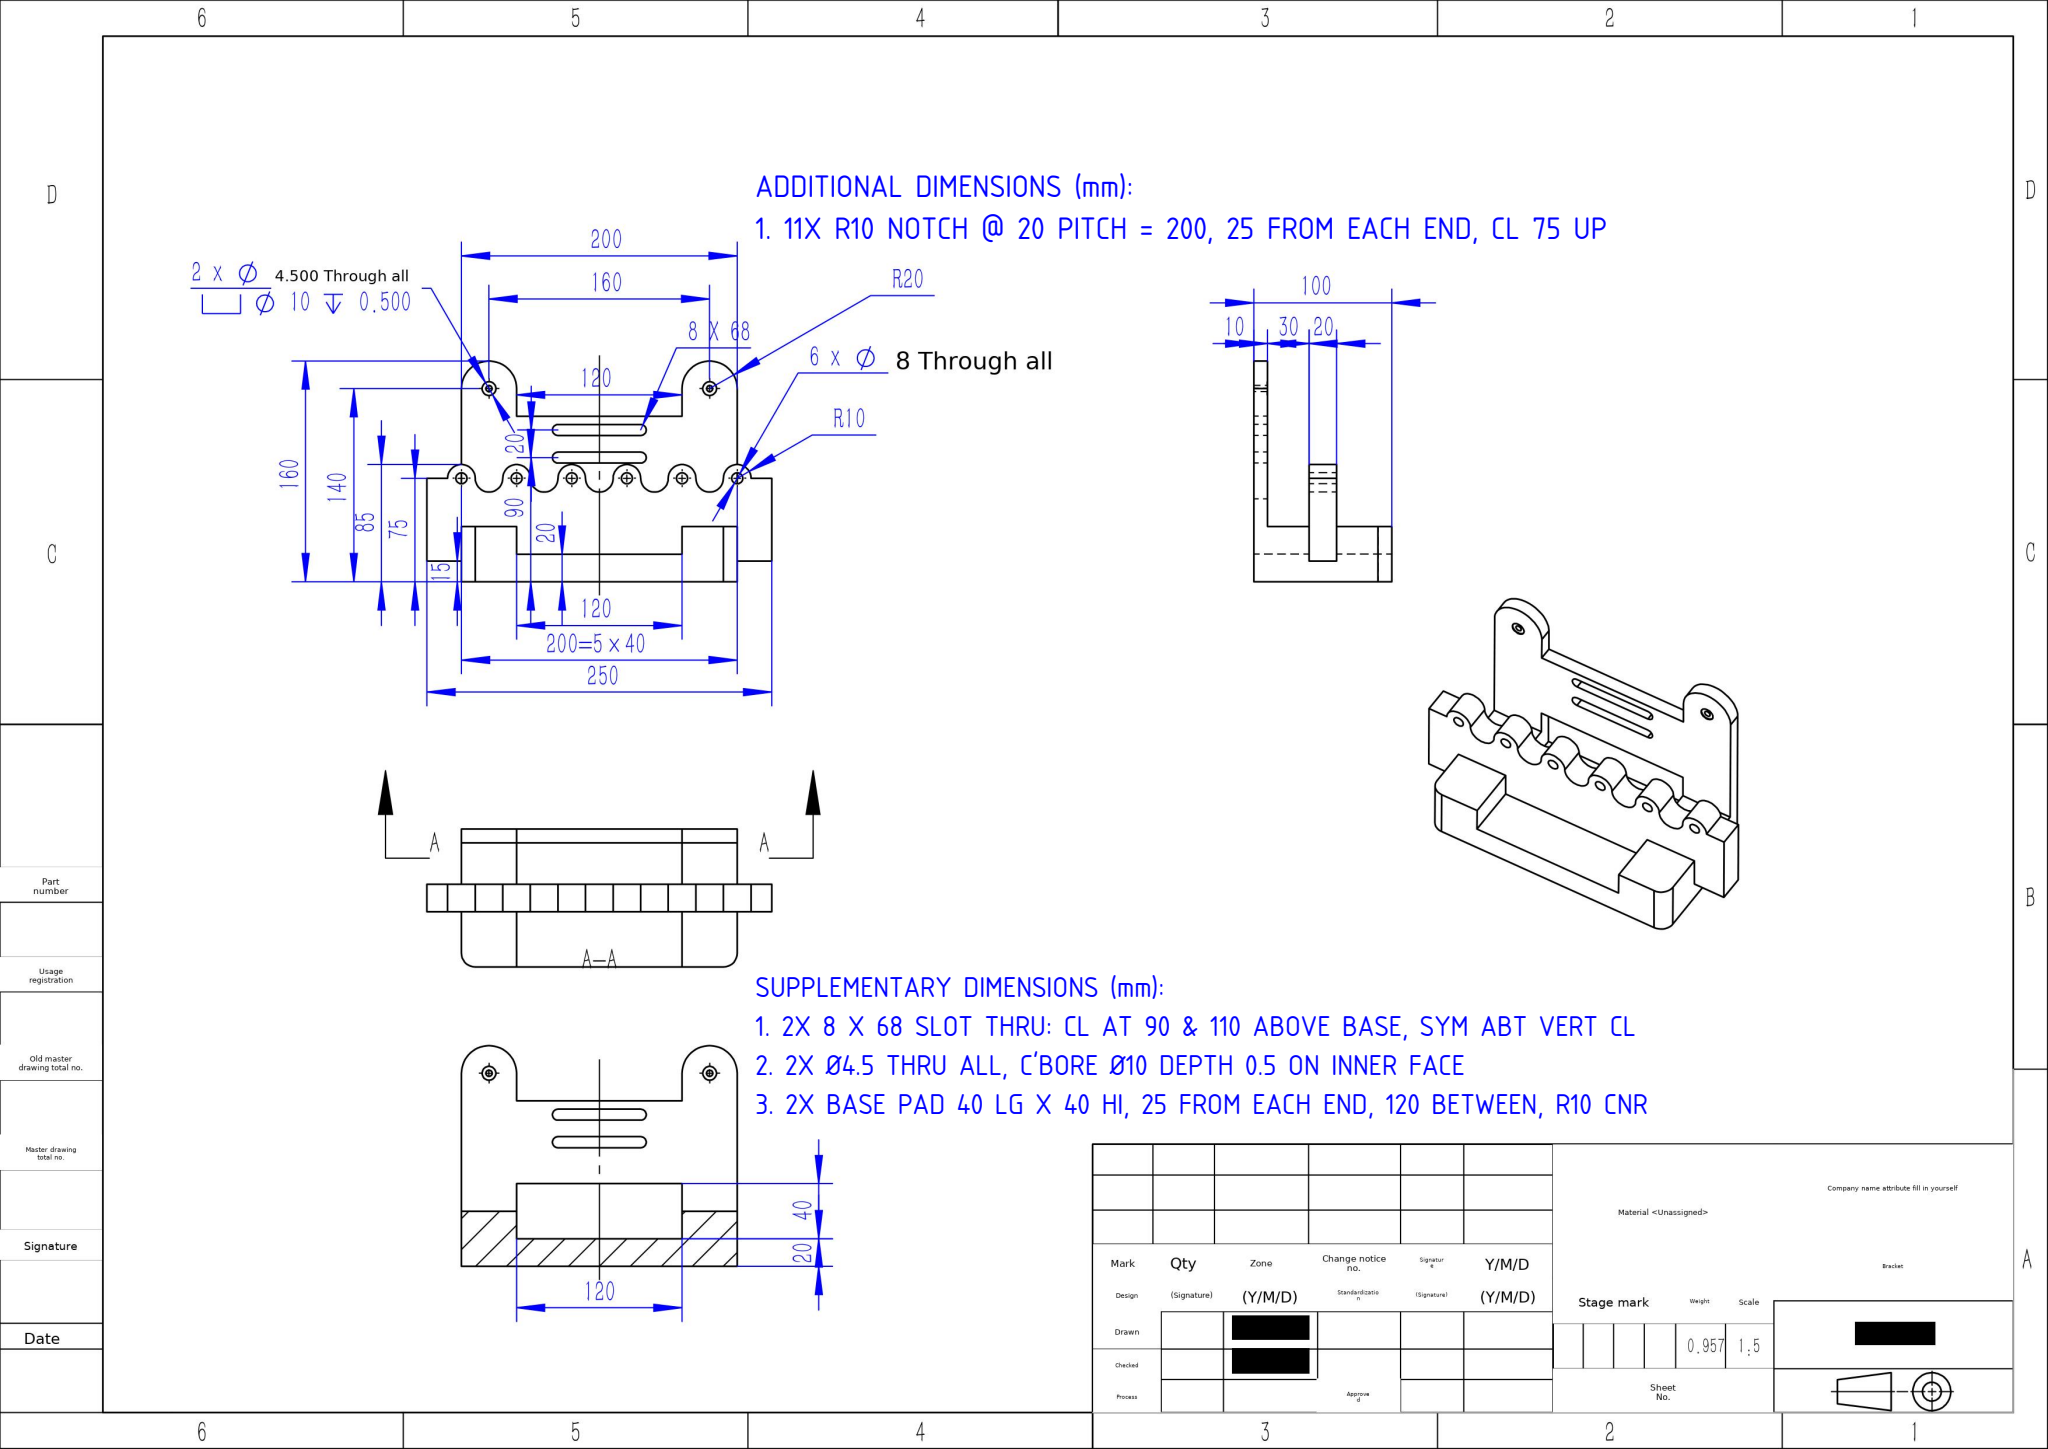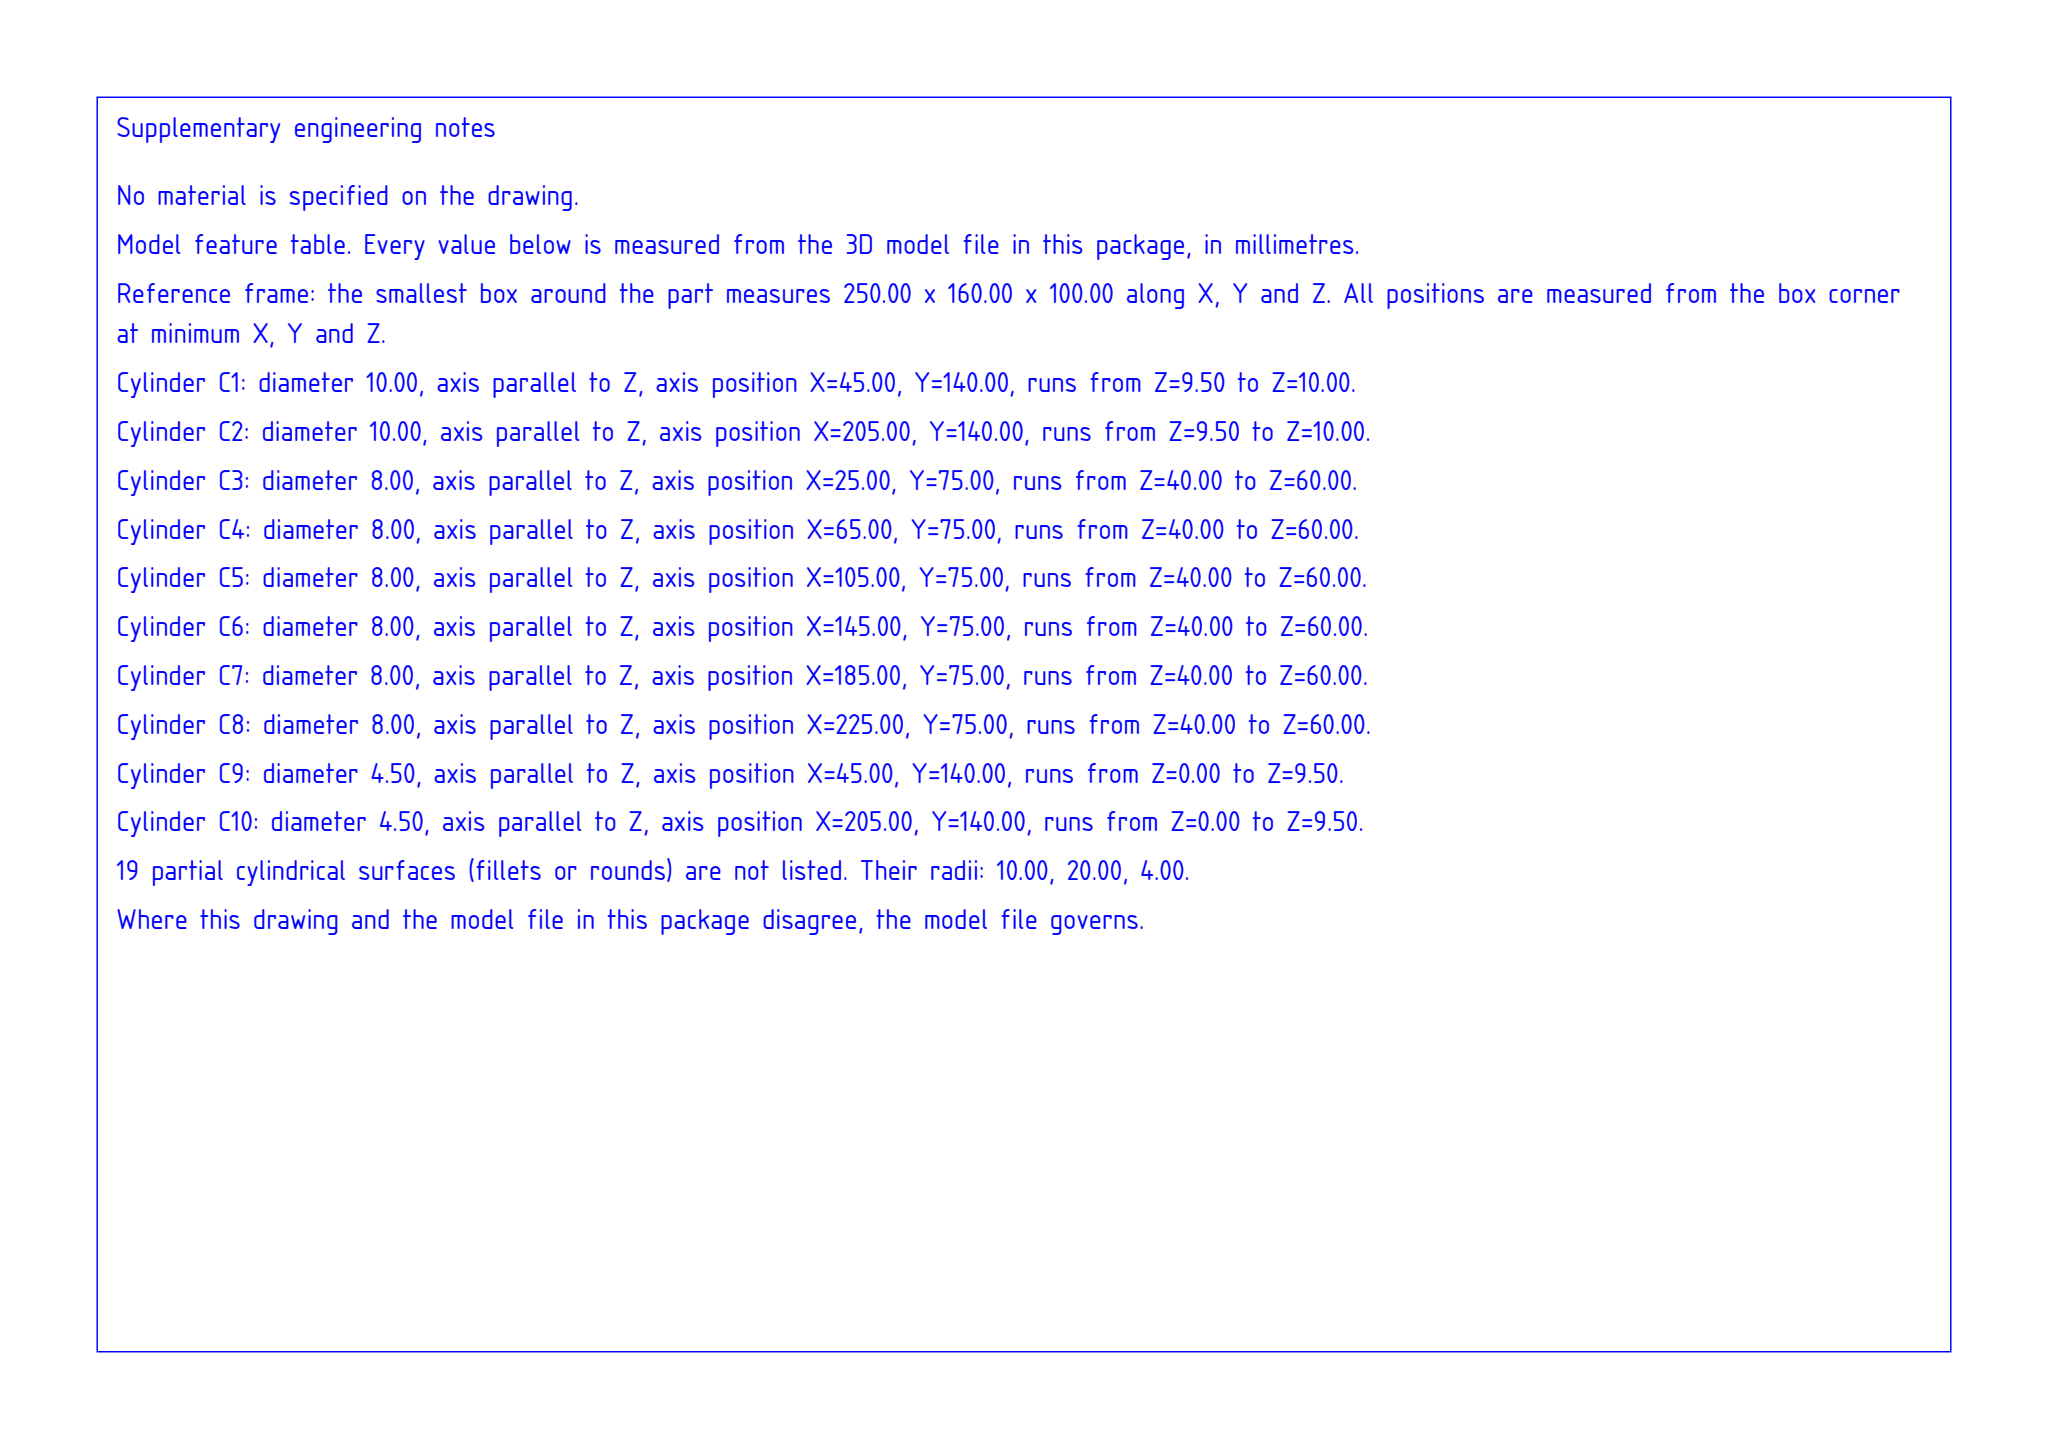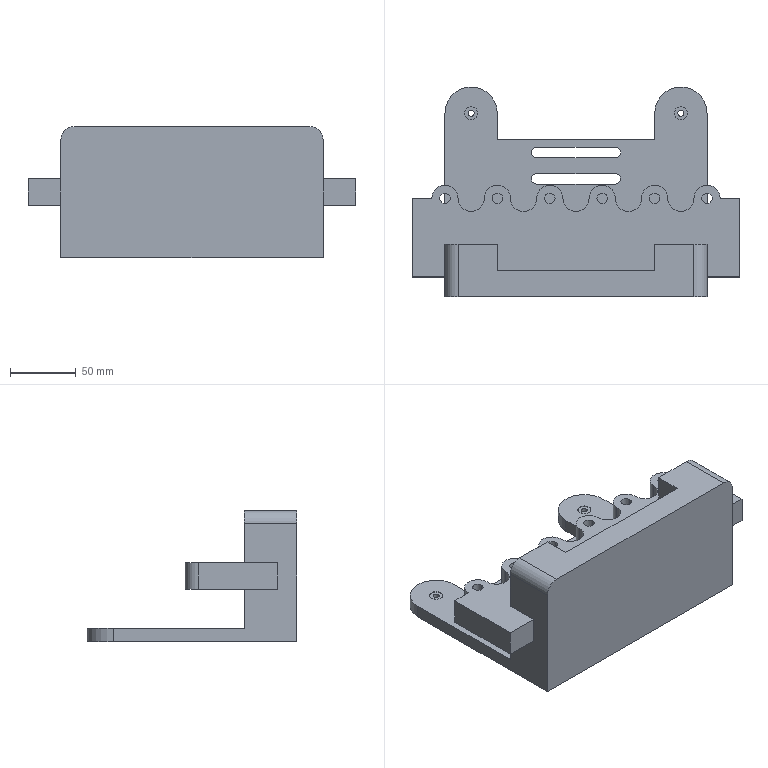Part | SolidWorks | mm | 1 solid | 75 faces | box 250 x 160 x 100 mm | volume 956973 mm3 | cylinder 41 | plane 34 | commonest cylinder face diameters 8 x18 20 x13 10 x4 4.5 x4 40 x2
build123d program:
from build123d import *

# Parameters (mm, degrees)
BOSS_EXTRUDE1_DEPTH                                 = 50
BOSS_EXTRUDE2_DEPTH                                 = 10
SKETCH3_R                                           = 10
CUT_EXTRUDE1_DEPTH                                  = 163.635
F_8_0_8_DIAMETER_HOLE1_D                            = 8
BOSS_EXTRUDE3_DEPTH                                 = 10
CYLINDRICAL_COUNTERSUNK_HOLE_FOR_M4_HEX_D           = 4.5
CYLINDRICAL_COUNTERSUNK_HOLE_FOR_M4_HEX_CBORE_D     = 10
CYLINDRICAL_COUNTERSUNK_HOLE_FOR_M4_HEX_CBORE_DEPTH = 0.5
FILLET1_R                                           = 10
CUT_EXTRUDE2_DEPTH                                  = 227.329


with BuildPart() as part:
    # Sketch1 → Boss-Extrude1 (new, symmetric)
    with BuildSketch(Plane.XY):
        Polygon((-60, 40), (-60, 20), (60, 20), (60, 40), (100, 40), (100, 0), (-100, 0), (-100, 40), align=None)
    extrude(amount=BOSS_EXTRUDE1_DEPTH, both=True)

    # Sketch2 → Boss-Extrude2 (add, symmetric)
    with BuildSketch(Plane.XY):
        with BuildLine():
            Line((-90, 75), (-70, 75))
            ThreePointArc((-70, 75), (-60, 85), (-50, 75))
            Line((-50, 75), (-30, 75))
            ThreePointArc((-30, 75), (-20, 85), (-10, 75))
            Line((-10, 75), (10, 75))
            ThreePointArc((10, 75), (20, 85), (30, 75))
            Line((30, 75), (50, 75))
            ThreePointArc((50, 75), (60, 85), (70, 75))
            Line((70, 75), (90, 75))
            ThreePointArc((90, 75), (100, 85), (110, 75))
            Line((110, 75), (125, 75))
            Line((125, 75), (125, 15))
            Line((125, 15), (100, 15))
            Line((100, 15), (100, 40))
            Line((100, 40), (60, 40))
            Line((60, 40), (60, 20))
            Line((60, 20), (-60, 20))
            Line((-60, 20), (-60, 40))
            Line((-60, 40), (-100, 40))
            Line((-100, 40), (-100, 15))
            Line((-100, 15), (-125, 15))
            Line((-125, 15), (-125, 75))
            Line((-125, 75), (-110, 75))
            ThreePointArc((-110, 75), (-100, 85), (-90, 75))
        make_face()
    extrude(amount=BOSS_EXTRUDE2_DEPTH, both=True)

    # Sketch3 → Cut-Extrude1 (cut, through all)
    with BuildSketch(Plane.XY.offset(10)):
        with Locations((-80, 75)):
            Circle(SKETCH3_R)
        with Locations((-40, 75)):
            Circle(SKETCH3_R)
        with Locations((0, 75)):
            Circle(SKETCH3_R)
        with Locations((40, 75)):
            Circle(SKETCH3_R)
        with Locations((80, 75)):
            Circle(SKETCH3_R)
    extrude(amount=-CUT_EXTRUDE1_DEPTH, mode=Mode.SUBTRACT)

    # 8.0 _8_ Diameter Hole1 (through all)
    with Locations(Plane.XY.offset(10)):
        with Locations((-100, 75), (-60, 75), (-20, 75), (20, 75), (60, 75), (100, 75)):
            Hole(F_8_0_8_DIAMETER_HOLE1_D / 2)

    # Sketch7 → Boss-Extrude3 (add)
    with BuildSketch(Plane(origin=(0, 0, -50), x_dir=(-1, 0, 0), z_dir=(0, 0, -1))):
        with BuildLine():
            Line((-100, 40), (-60, 40))
            Line((-60, 40), (-60, 60))
            Line((-60, 60), (60, 60))
            Line((60, 60), (60, 40))
            Line((60, 40), (100, 40))
            Line((100, 40), (100, 140))
            ThreePointArc((100, 140), (80, 160), (60, 140))
            Line((60, 140), (60, 120))
            Line((60, 120), (-60, 120))
            Line((-60, 120), (-60, 140))
            ThreePointArc((-60, 140), (-80, 160), (-100, 140))
            Line((-100, 140), (-100, 40))
        make_face()
    extrude(amount=-BOSS_EXTRUDE3_DEPTH)

    # Cylindrical Countersunk Hole for M4 Hex (through all)
    with Locations(Plane.XY.offset(-40)):
        with Locations((-80, 140), (80, 140)):
            CounterBoreHole(CYLINDRICAL_COUNTERSUNK_HOLE_FOR_M4_HEX_D / 2, CYLINDRICAL_COUNTERSUNK_HOLE_FOR_M4_HEX_CBORE_D / 2, CYLINDRICAL_COUNTERSUNK_HOLE_FOR_M4_HEX_CBORE_DEPTH)

    # Fillet1
    fillet1_edges = [part.edges().sort_by_distance(p)[0] for p in [
        (100, 20, 50),
        (-100, 20, 50),
    ]]
    fillet(fillet1_edges, radius=FILLET1_R)

    # Sketch11 → Cut-Extrude2 (cut, through all)
    with BuildSketch(Plane(origin=(0, 0, -50), x_dir=(-1, 0, 0), z_dir=(0, 0, -1))):
        with BuildLine():
            Line((-30, 114), (30, 114))
            ThreePointArc((30, 114), (34, 110), (30, 106))
            Line((30, 106), (-30, 106))
            ThreePointArc((-30, 106), (-34, 110), (-30, 114))
        make_face()
        with BuildLine():
            Line((-30, 94), (30, 94))
            ThreePointArc((30, 94), (34, 90), (30, 86))
            Line((30, 86), (-30, 86))
            ThreePointArc((-30, 86), (-34, 90), (-30, 94))
        make_face()
    extrude(amount=-CUT_EXTRUDE2_DEPTH, mode=Mode.SUBTRACT)


solid = part.part